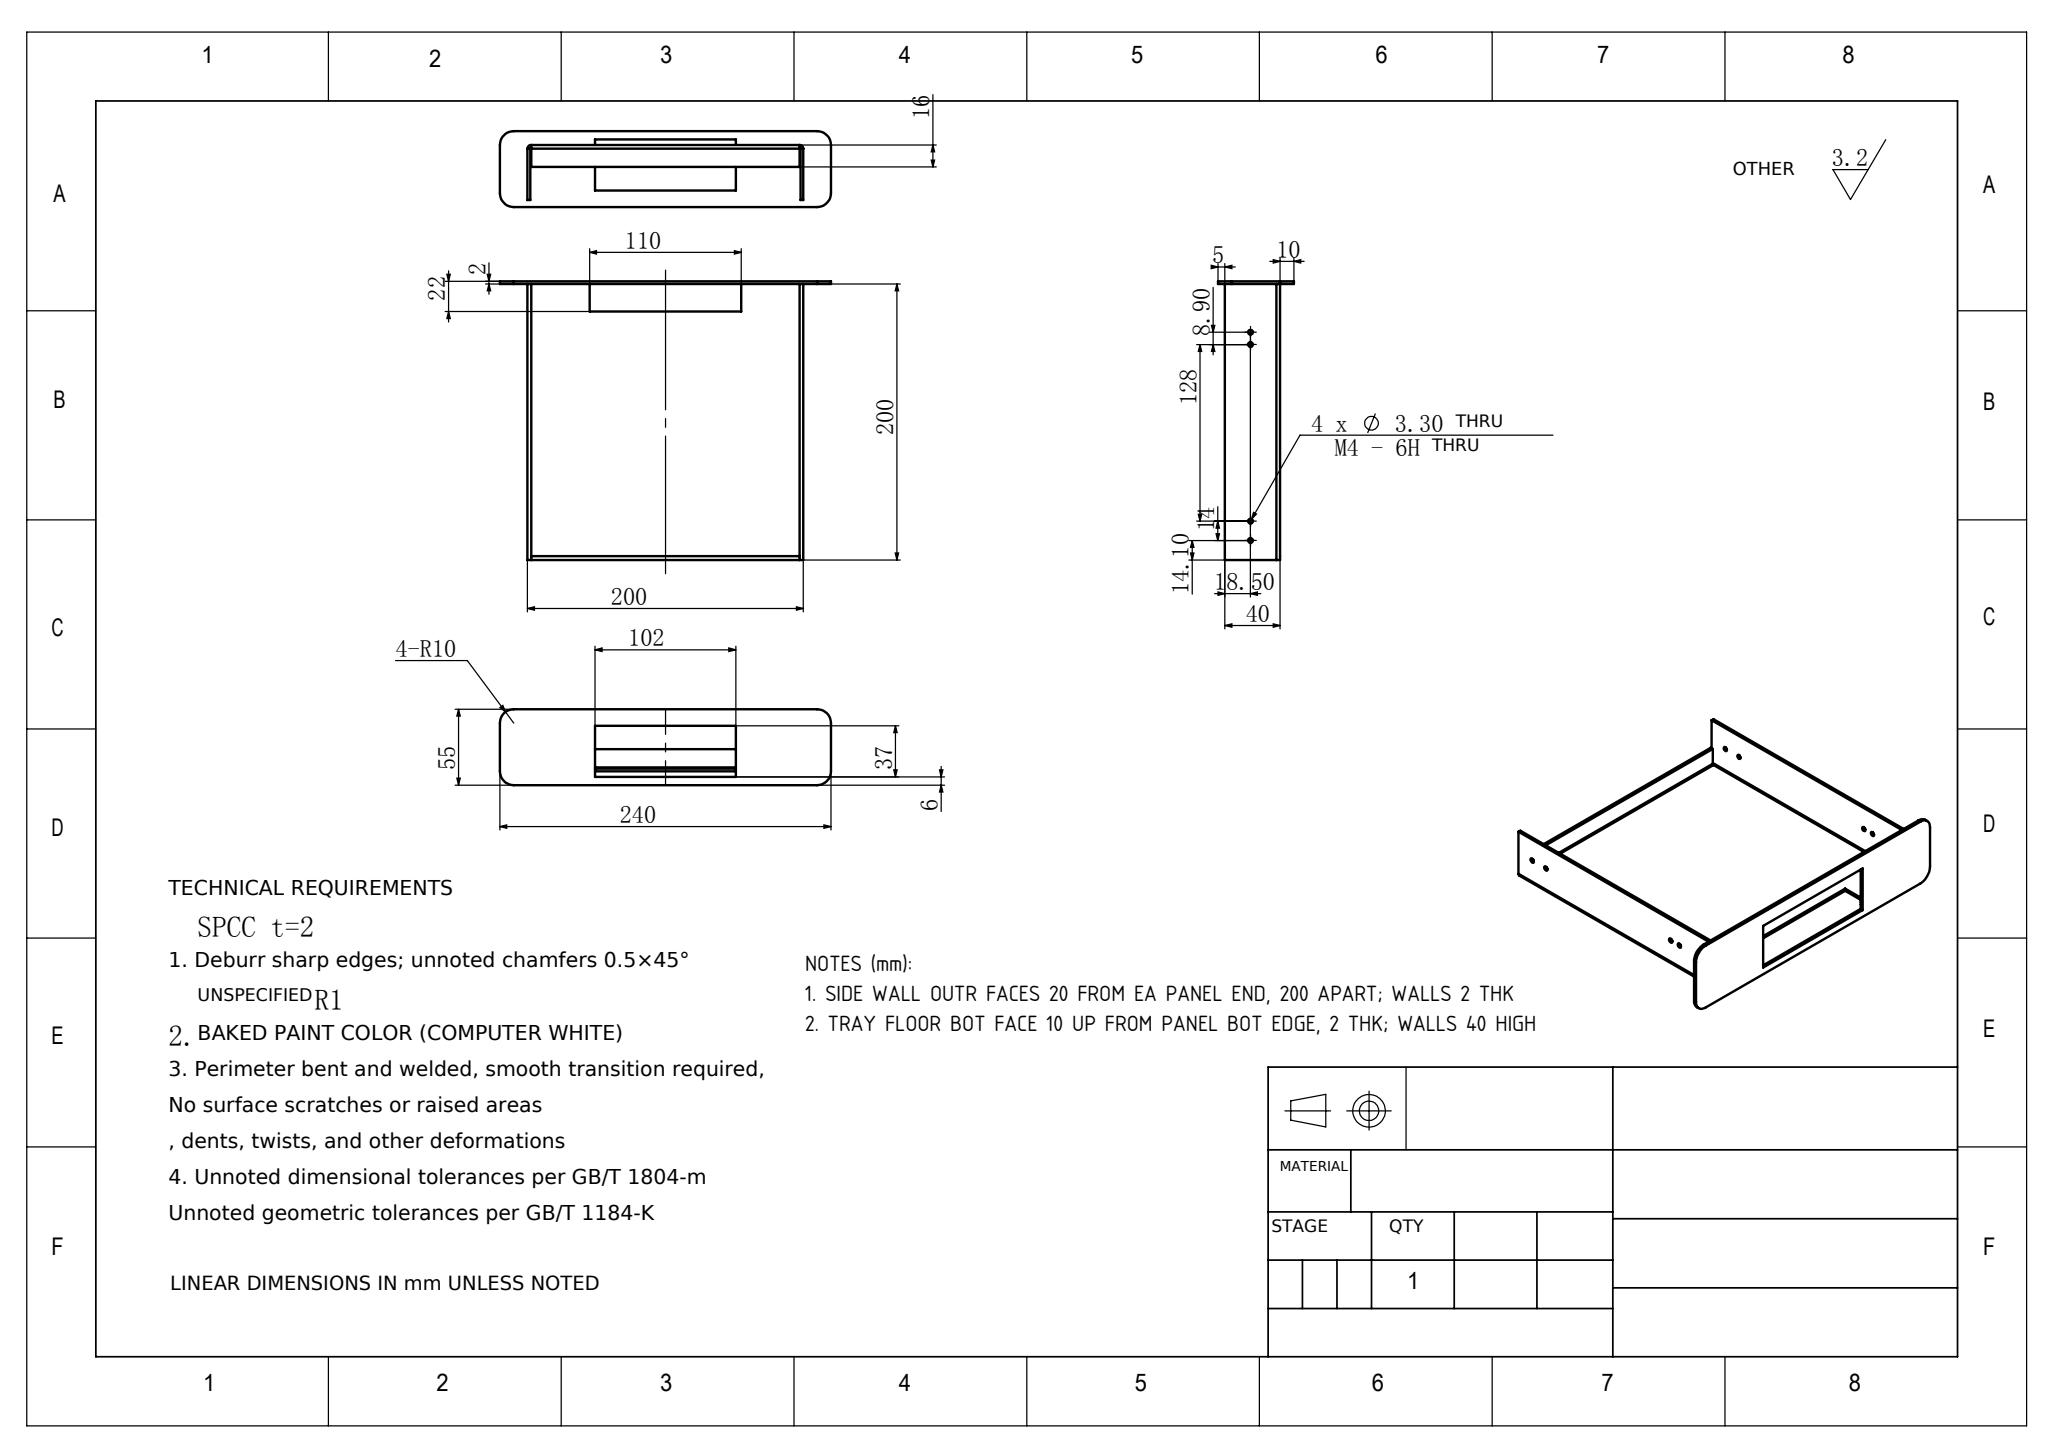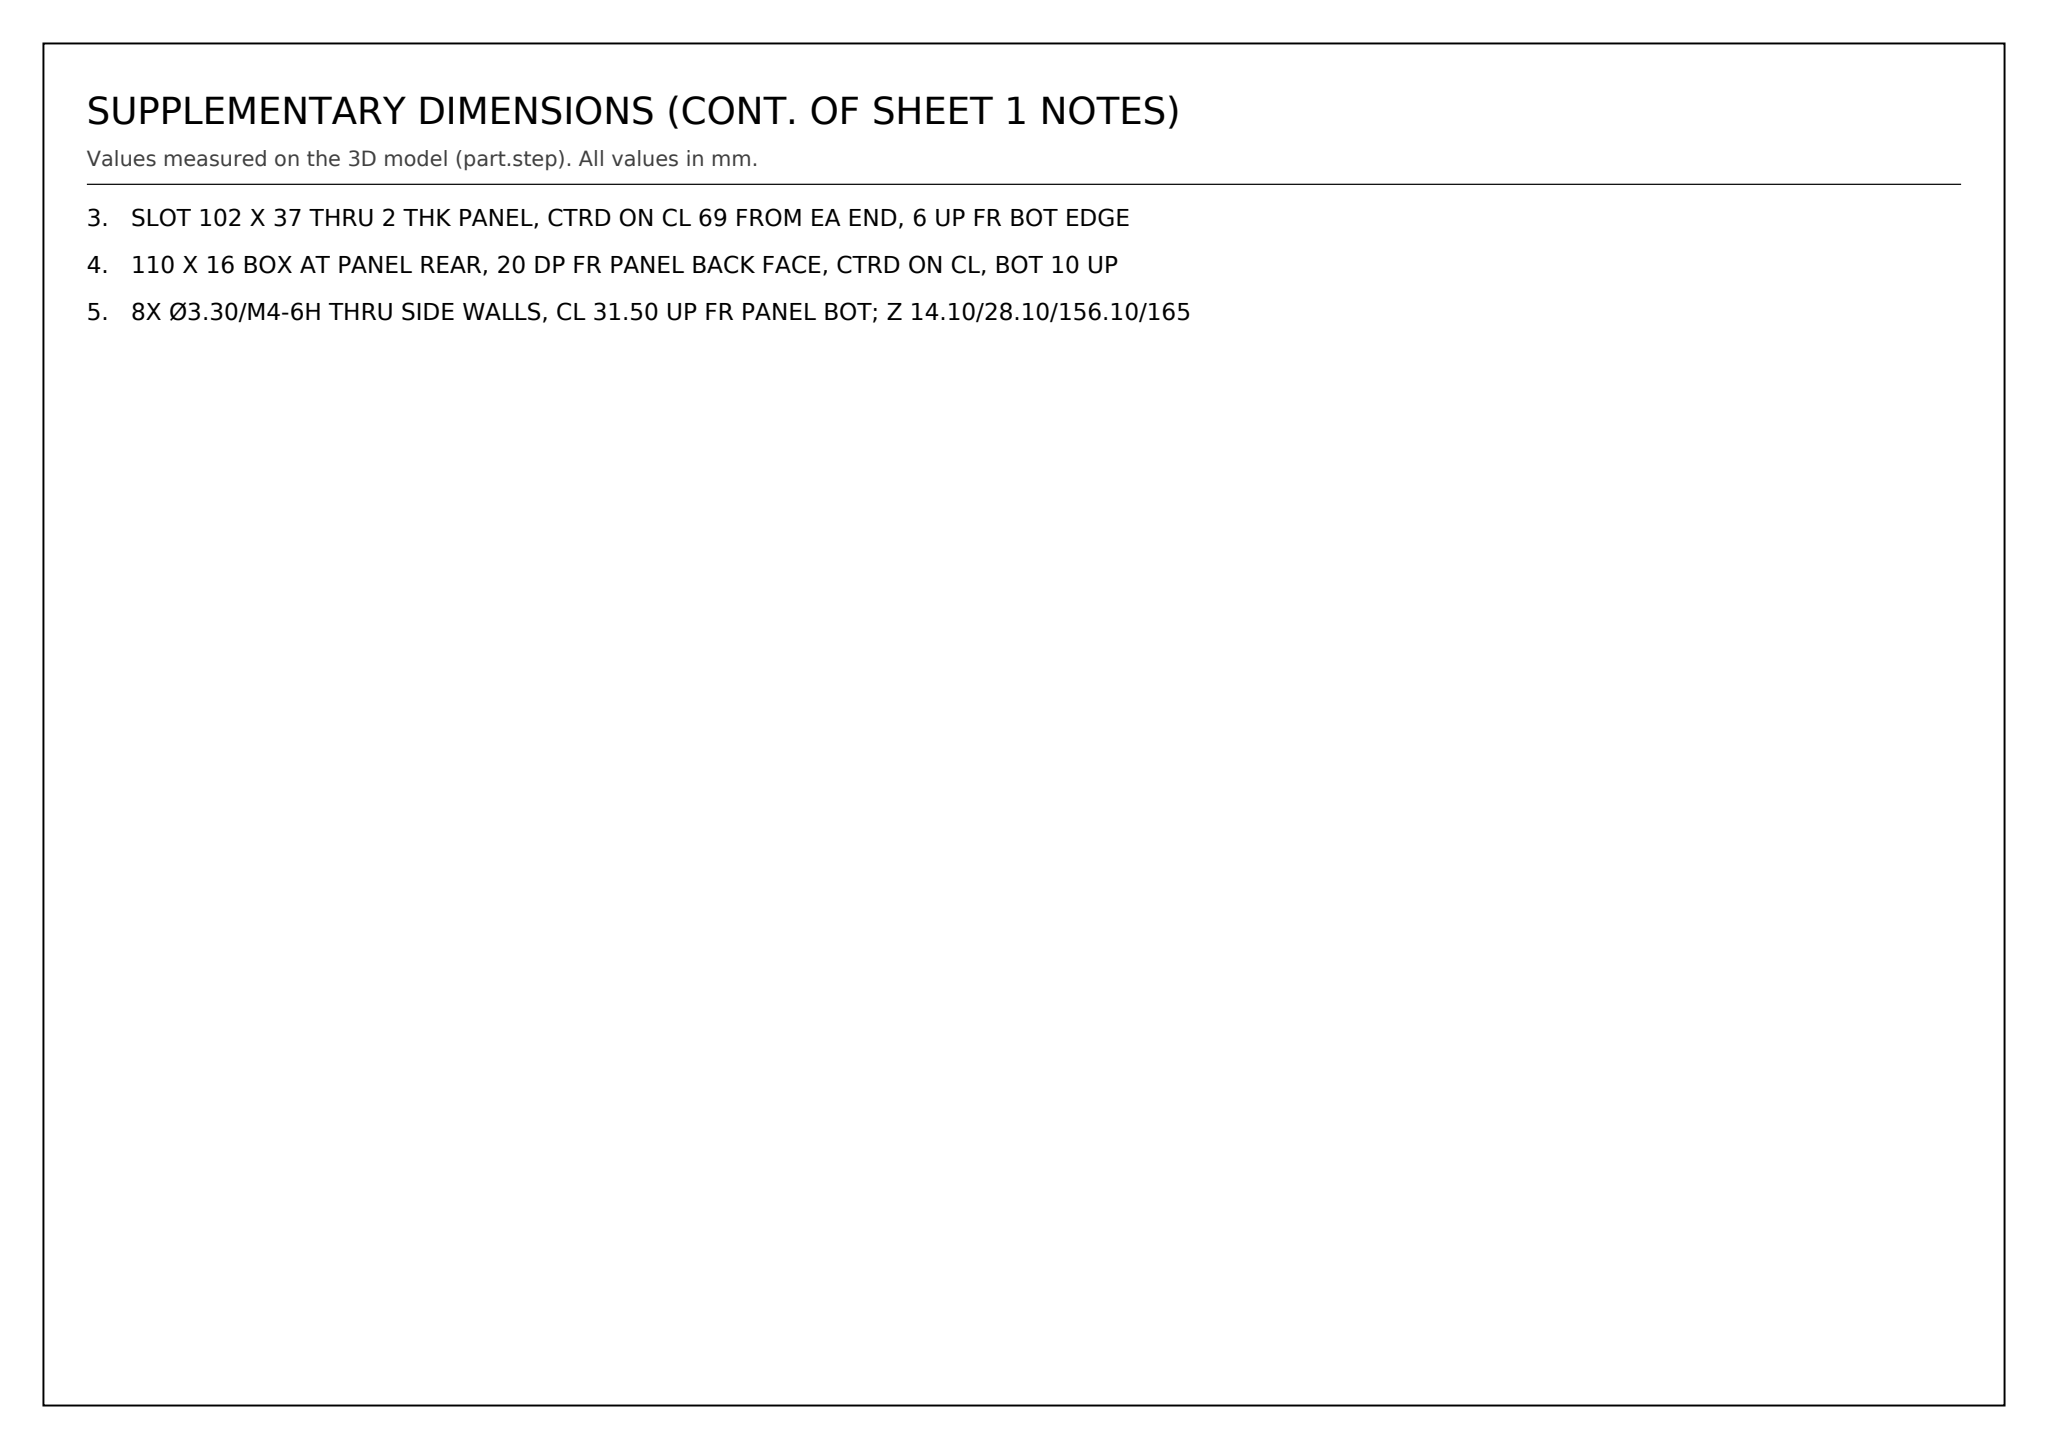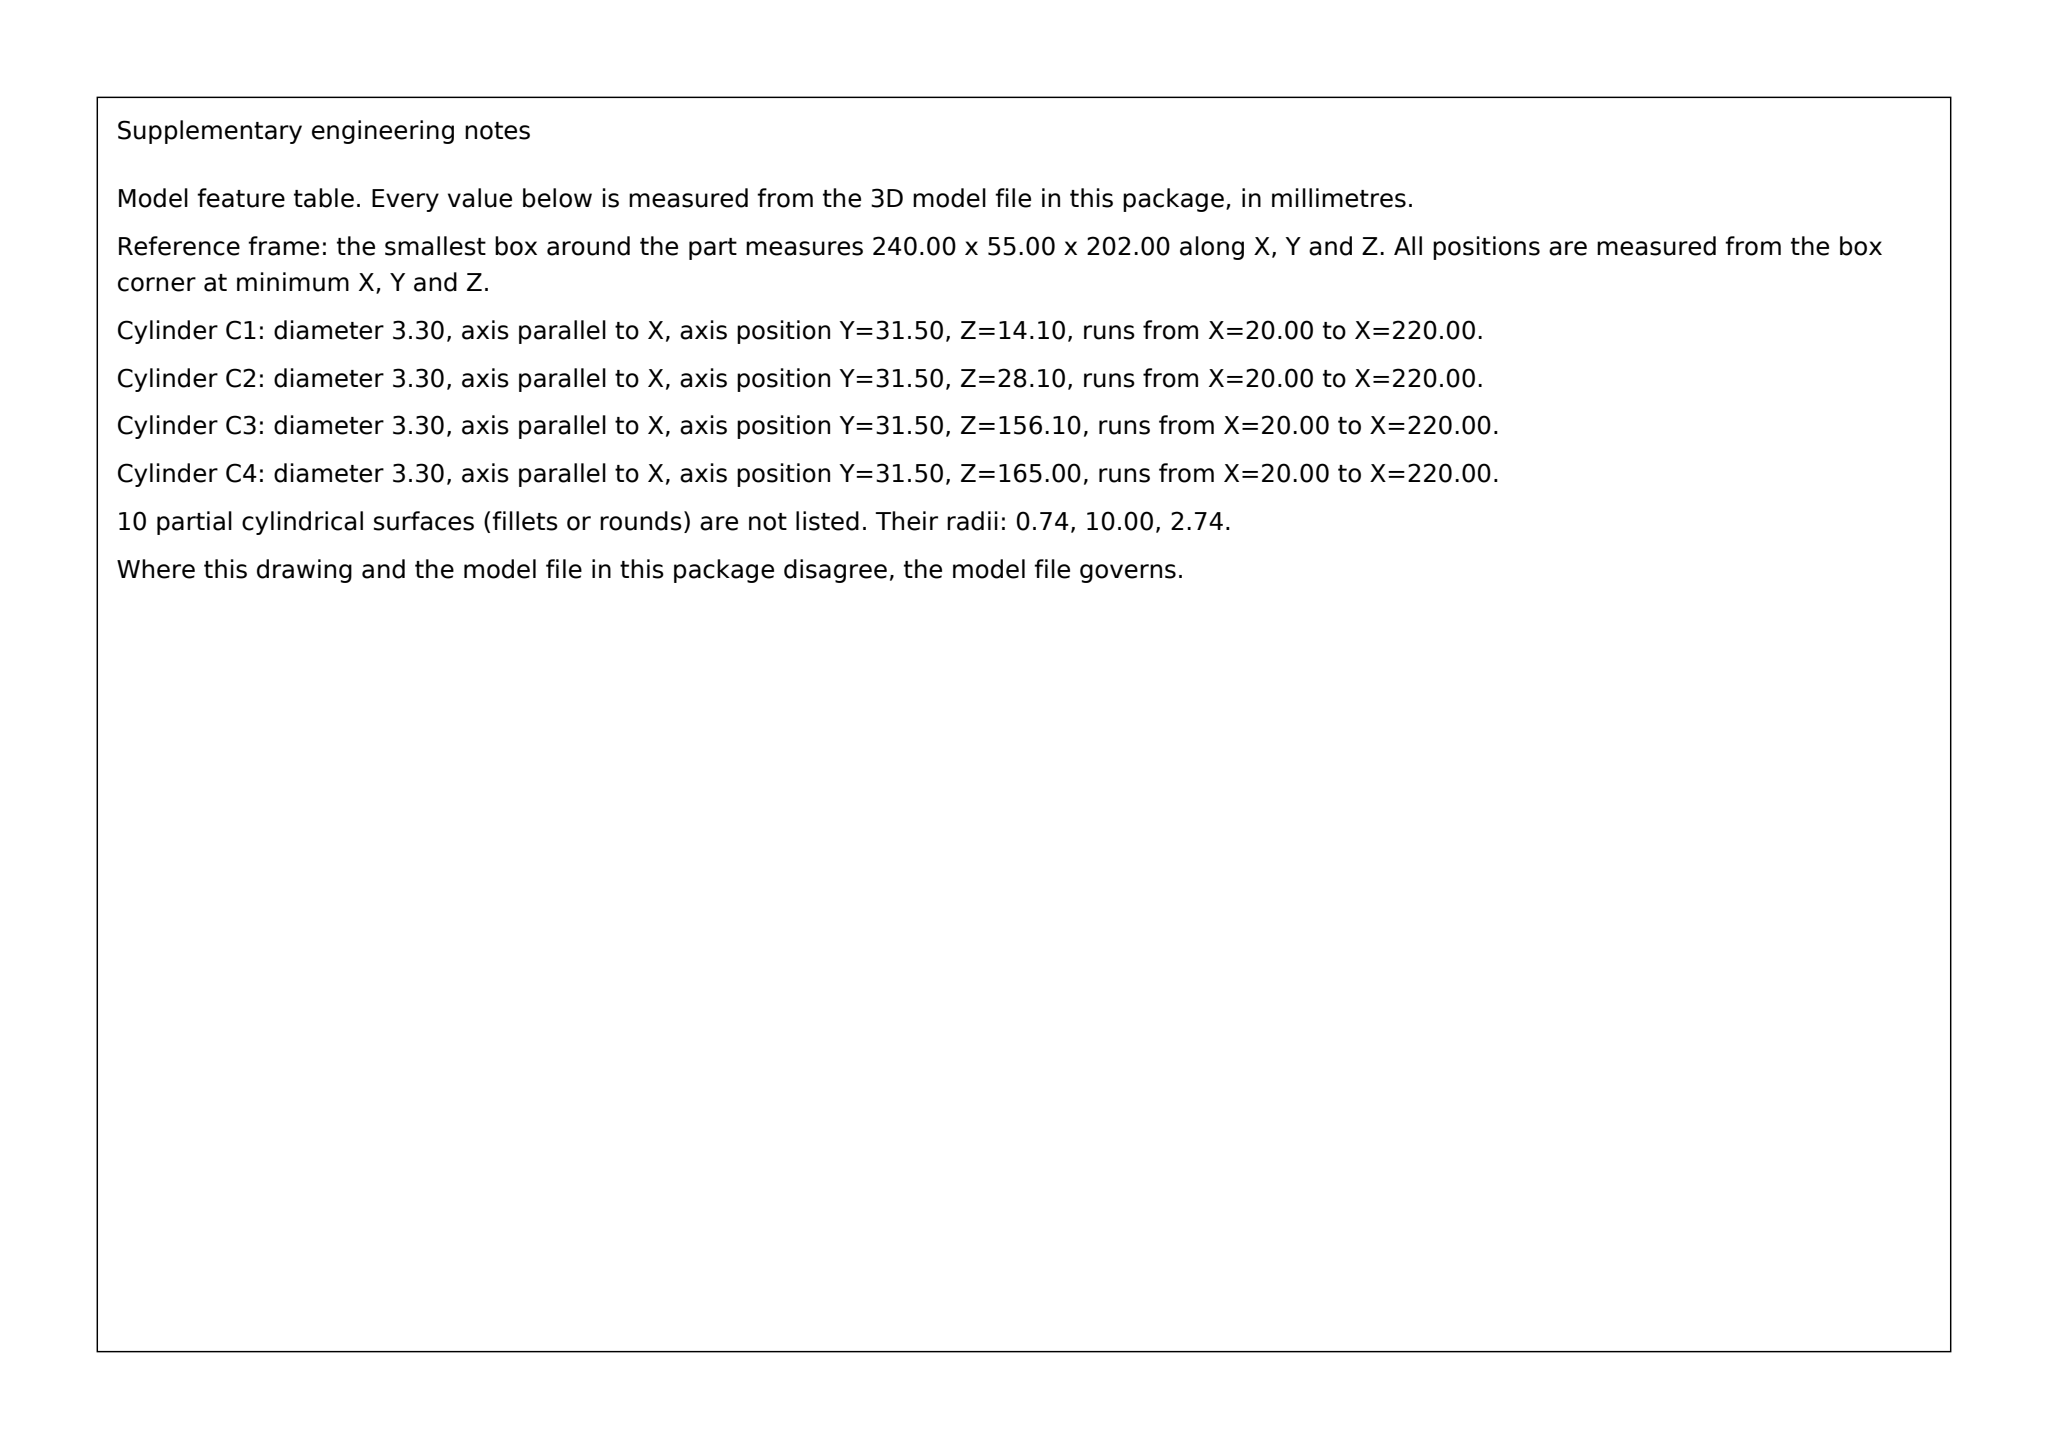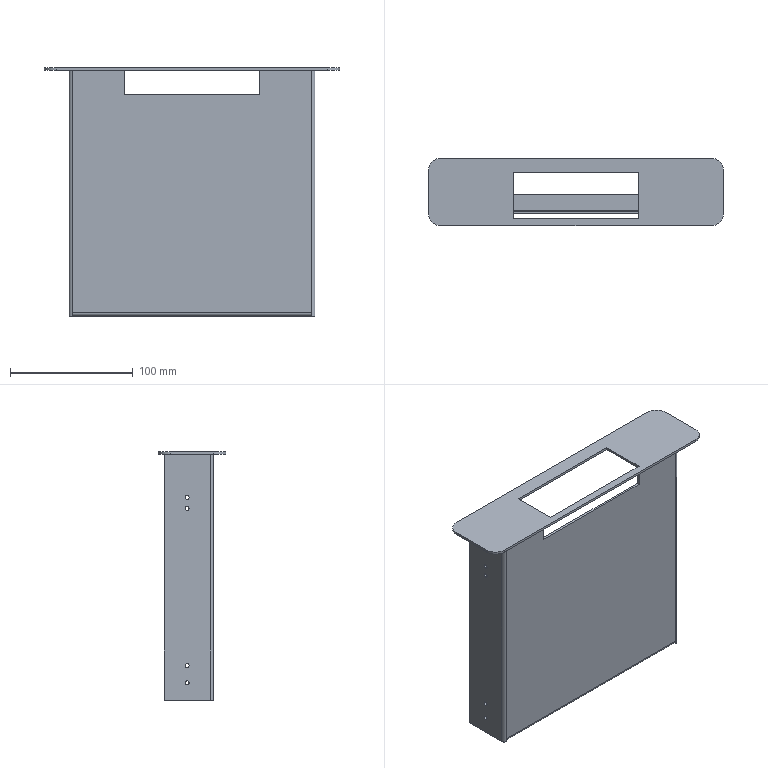Part | SolidWorks | mm | 1 solid | 62 faces | box 240 x 55 x 202 mm | volume 129104 mm3 | plane 36 | cylinder 26 | commonest cylinder face diameters 3.3 x16 20 x4 5.473 x3 1.473 x3
Drawing notes:
SIDE WALL OUTR FACES 20 FROM EA PANEL END, 200 APART; WALLS 2 THK | from the solid: x planes 20.0, 22.0, 218.0, 220.0 in 240 wide bbox
TRAY FLOOR BOT FACE 10 UP FROM PANEL BOT EDGE, 2 THK; WALLS 40 HIGH | from the solid: y planes 0 (panel bot), 10/12 (floor 2 thk), 50 (wall top): 50-10=40
SLOT 102 X 37 THRU 2 THK PANEL, CTRD ON CL 69 FROM EA END, 6 UP FR BOT EDGE | from the solid: slot x 69..171 in 240 wide panel, y 6..43, panel z 0..2
110 X 16 BOX AT PANEL REAR, 20 DP FR PANEL BACK FACE, CTRD ON CL, BOT 10 UP | from the solid: x 65/175 ctr 120, y 10/26, z 180 to 200 back face; 22 incl 2 thk panel
8X Ø3.30/M4-6H THRU SIDE WALLS, CL 31.50 UP FR PANEL BOT; Z 14.10/28.10/156.10/165 | from the solid: Ø3.3 cyl axis X len 2.0 at y=31.5, z=14.1/28.1/156.1/165, walls x20-22 & x218-220; 50-31.5=18.50